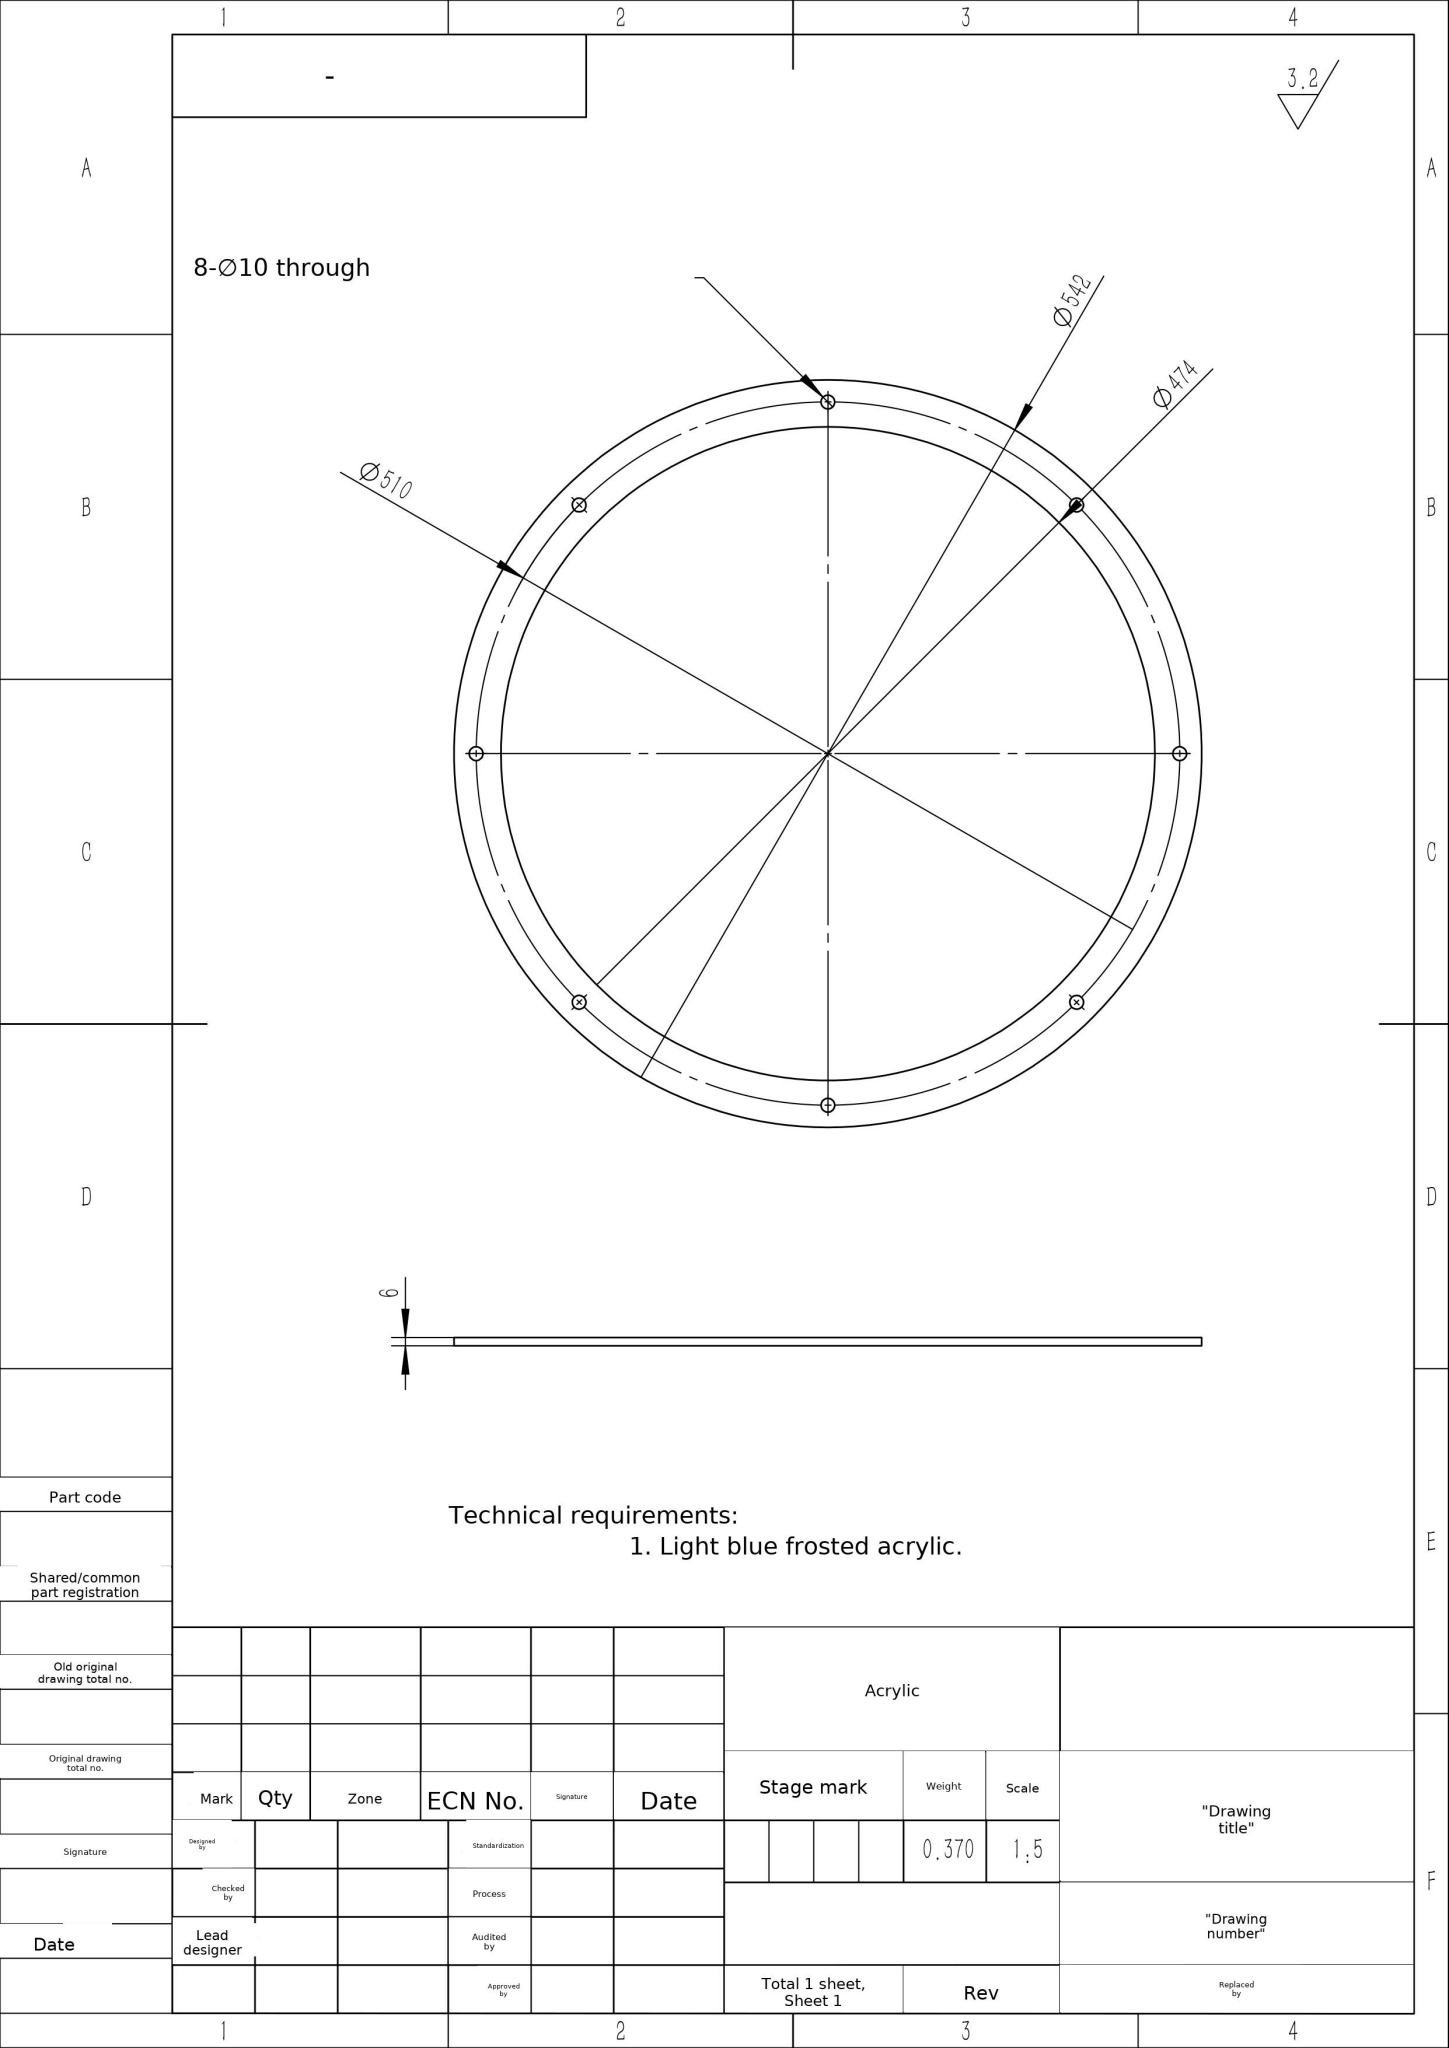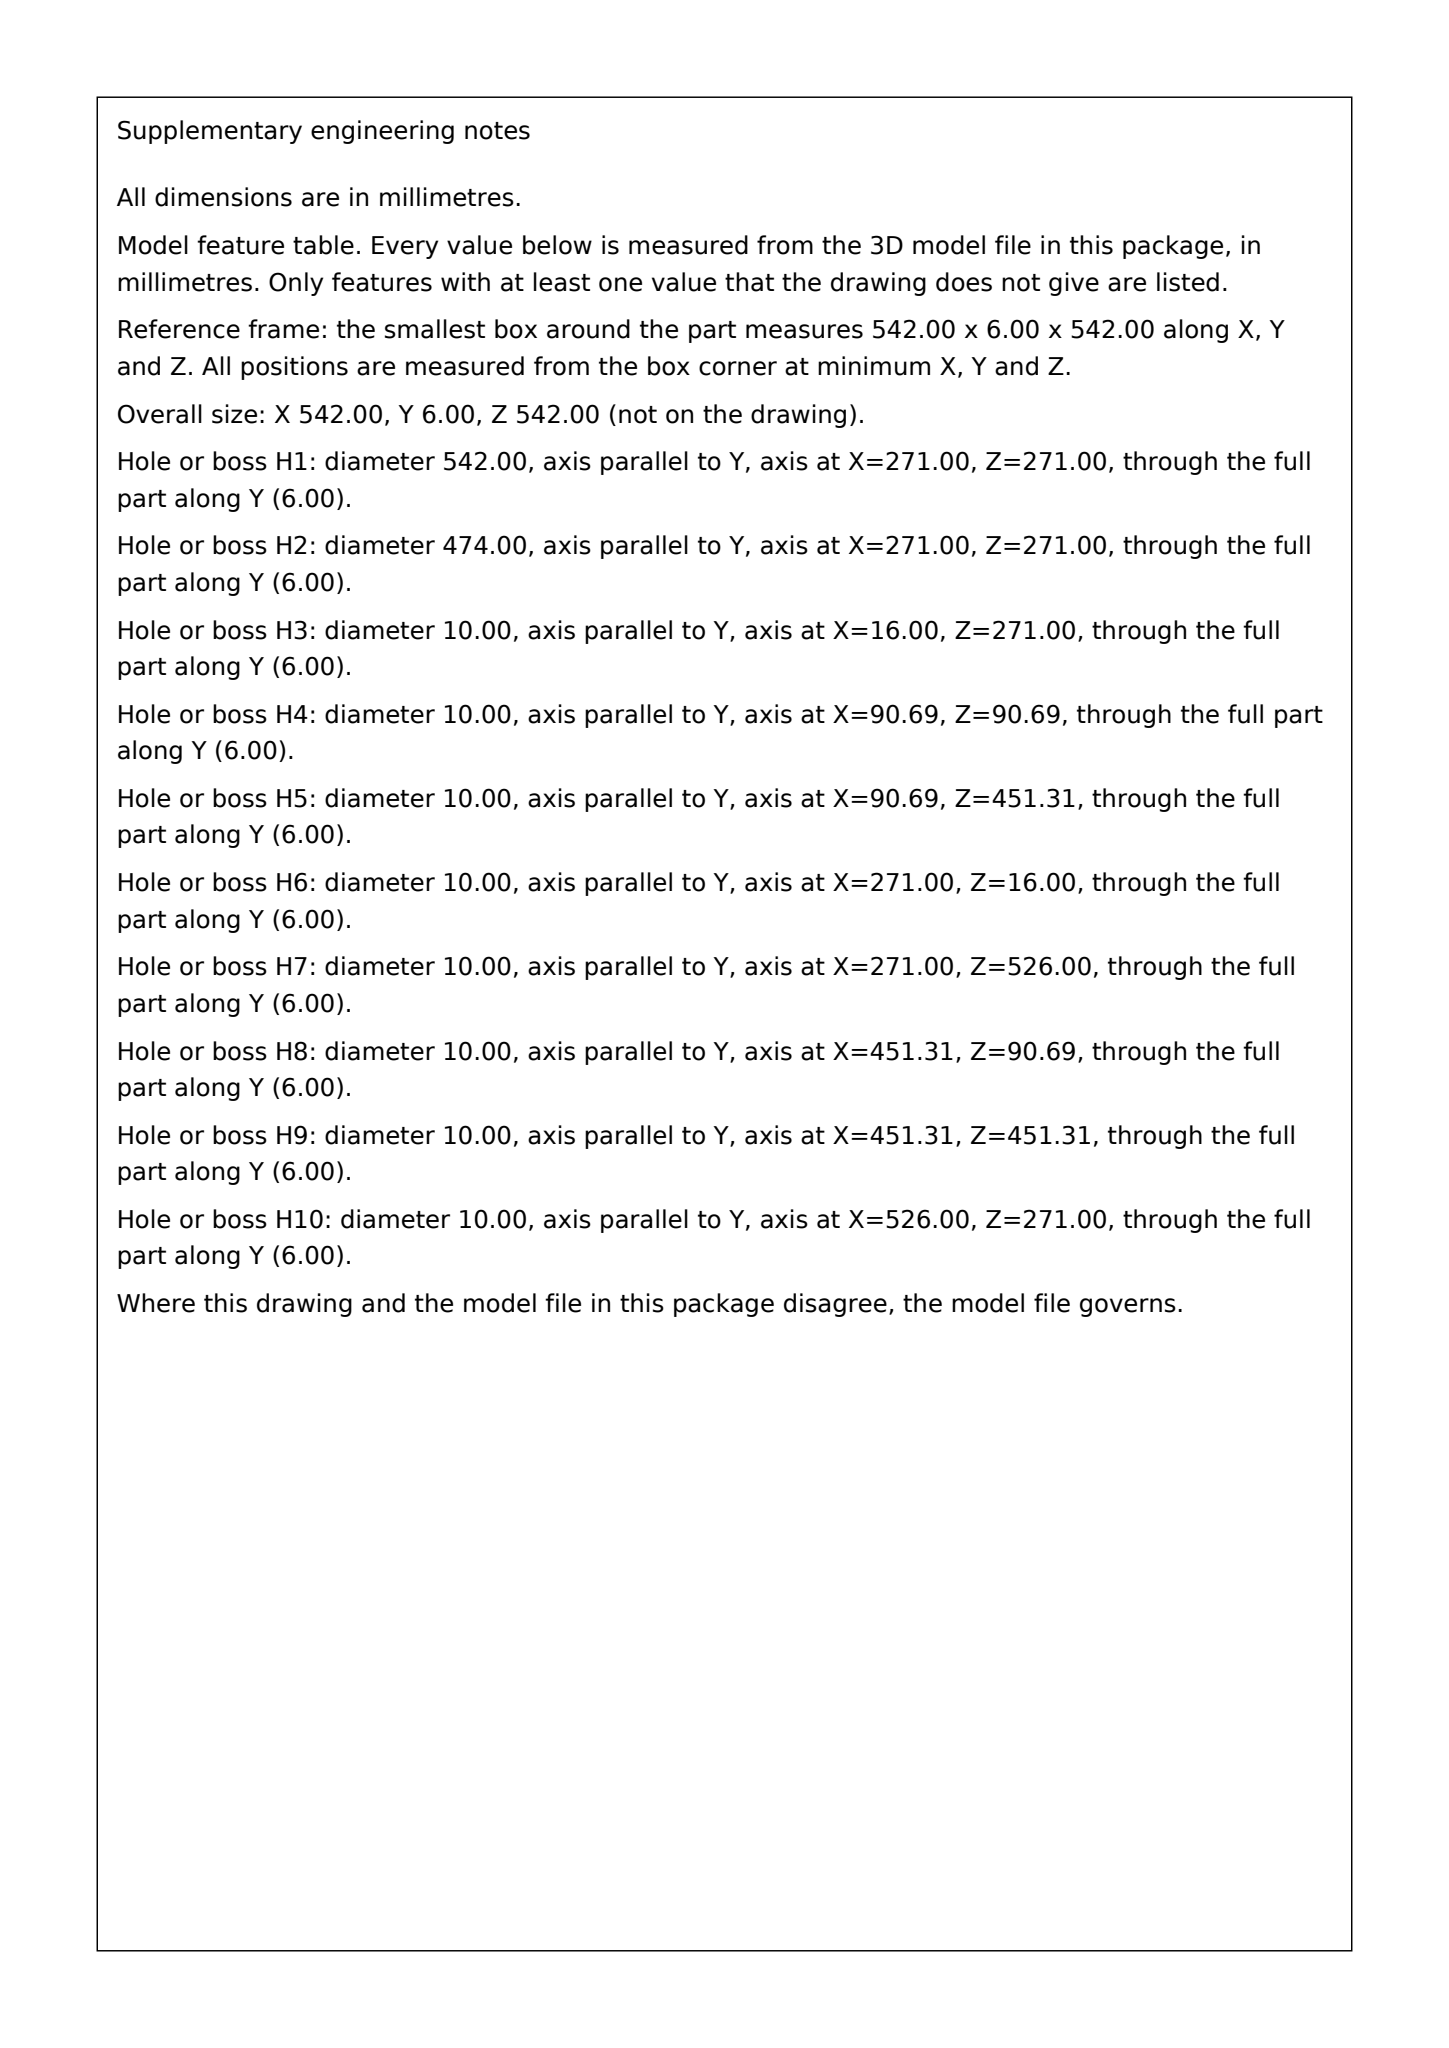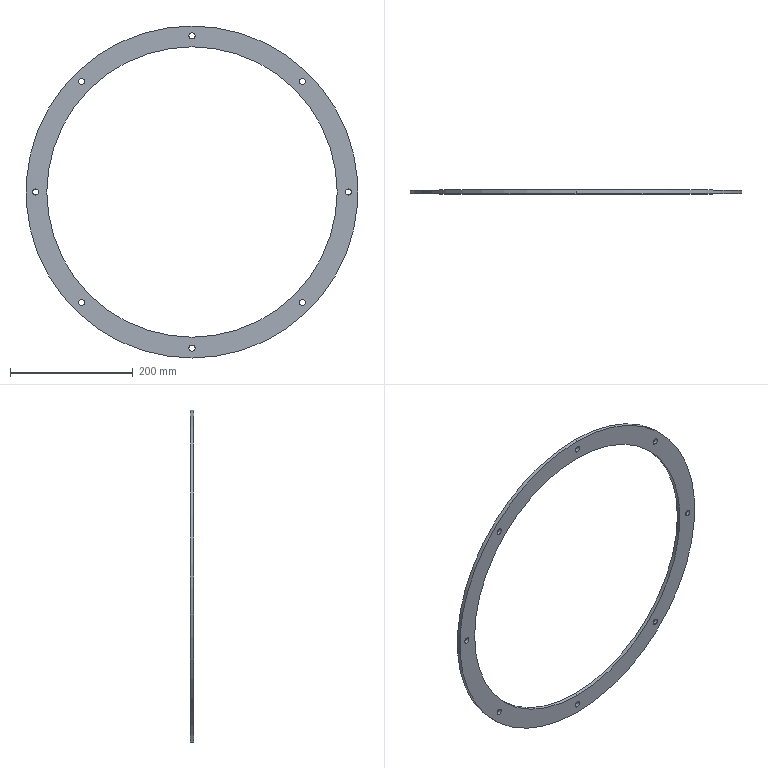Part | SolidWorks | mm | material Acrylic | 1 solid | 22 faces | box 542 x 6 x 542 mm | volume 321800 mm3 | cylinder 20 | plane 2 | commonest cylinder face diameters 10 x16 542 x2 474 x2
build123d program:
from build123d import *

# Parameters (mm, degrees)
SKETCH1_W          = 34
SKETCH1_H          = 3
SKETCH2_R          = 5
CUT_EXTRUDE1_DEPTH = 30
CIRPATTERN1_COUNT  = 8


with BuildPart() as part:
    # Sketch1 → Revolve1 (revolve)
    with BuildSketch(Plane.XY, mode=Mode.PRIVATE) as revolve1_sk:
        with Locations((254, 1.5)):
            Rectangle(SKETCH1_W, SKETCH1_H)
    revolve1 = revolve(revolve1_sk.sketch.rotate(Axis((0, 0, 0), (0, 1, 0)), 90), axis=Axis((0, 0, 0), (0, 1, 0)))


with BuildPart() as mirror1_1:
    # Mirror1: Revolve1 across Top Plane
    add(revolve1.mirror(Plane(origin=(0, 0, 0), x_dir=(1, 0, 0), z_dir=(0, 1, 0))))


with BuildPart() as part_1:
    add(part.part)

    # Mirror1 united with what the copies touc: union Mirror1_1
    add(mirror1_1.part)

    # Sketch2 → Cut-Extrude1 (cut)
    with BuildSketch(Plane(origin=(0, 3, 0), x_dir=(1, 0, 0), z_dir=(0, 1, 0))):
        with Locations(Location((255, 0, 0), (0, 0, 270))):
            Circle(SKETCH2_R)
    cut_extrude1 = extrude(amount=-CUT_EXTRUDE1_DEPTH, mode=Mode.SUBTRACT)

    # CirPattern1: Cut-Extrude1 ×8 about axis
    cirpattern1_axis = Axis((0, 0, 0), (0, 1, 0))
    for i in range(1, CIRPATTERN1_COUNT):
        add(cut_extrude1.rotate(cirpattern1_axis, i * 360 / CIRPATTERN1_COUNT), mode=Mode.SUBTRACT)


solid = part_1.part
STEP:
#1=CARTESIAN_POINT('',(-0.,-3.,250.));
#2=VERTEX_POINT('',#1);
#3=CARTESIAN_POINT('',(-0.,-3.,260.));
#4=VERTEX_POINT('',#3);
#5=CARTESIAN_POINT('',(-0.,-3.,255.));
#6=DIRECTION('',(0.,1.,0.));
#7=DIRECTION('',(0.,0.,1.));
#8=AXIS2_PLACEMENT_3D('',#5,#6,#7);
#9=CIRCLE('',#8,5.);
#10=EDGE_CURVE('',#2,#4,#9,.T.);
#11=ORIENTED_EDGE('',*,*,#10,.F.);
#12=CARTESIAN_POINT('',(-0.,3.,250.));
#13=VERTEX_POINT('',#12);
#14=CARTESIAN_POINT('',(-0.,-27.,250.));
#15=DIRECTION('',(0.,1.,0.));
#16=VECTOR('',#15,1000.);
#17=LINE('',#14,#16);
#18=EDGE_CURVE('',#2,#13,#17,.T.);
#19=ORIENTED_EDGE('',*,*,#18,.T.);
#20=CARTESIAN_POINT('',(-0.,3.,260.));
#21=VERTEX_POINT('',#20);
#22=CARTESIAN_POINT('',(-0.,3.,255.));
#23=DIRECTION('',(0.,1.,0.));
#24=DIRECTION('',(-1.,0.,0.));
#25=AXIS2_PLACEMENT_3D('',#22,#23,#24);
#26=CIRCLE('',#25,5.);
#27=EDGE_CURVE('',#13,#21,#26,.T.);
#28=ORIENTED_EDGE('',*,*,#27,.T.);
#29=CARTESIAN_POINT('',(-0.,-27.,260.));
#30=DIRECTION('',(0.,1.,0.));
#31=VECTOR('',#30,1000.);
#32=LINE('',#29,#31);
#33=EDGE_CURVE('',#4,#21,#32,.T.);
#34=ORIENTED_EDGE('',*,*,#33,.F.);
#35=EDGE_LOOP('',(#11,#19,#28,#34));
#36=FACE_OUTER_BOUND('',#35,.T.);
#37=CARTESIAN_POINT('',(-0.,-27.,255.));
#38=DIRECTION('',(0.,1.,0.));
#39=DIRECTION('',(0.,0.,1.));
#40=AXIS2_PLACEMENT_3D('',#37,#38,#39);
#41=CYLINDRICAL_SURFACE('',#40,5.);
#42=ADVANCED_FACE('',(#36),#41,.F.);
#43=CARTESIAN_POINT('',(-180.312,-3.,175.312));
#44=VERTEX_POINT('',#43);
#45=CARTESIAN_POINT('',(-180.312,-3.,185.312));
#46=VERTEX_POINT('',#45);
#47=CARTESIAN_POINT('',(-180.312,-3.,180.312));
#48=DIRECTION('',(0.,1.,0.));
#49=DIRECTION('',(0.,0.,1.));
#50=AXIS2_PLACEMENT_3D('',#47,#48,#49);
#51=CIRCLE('',#50,5.);
#52=EDGE_CURVE('',#44,#46,#51,.T.);
#53=ORIENTED_EDGE('',*,*,#52,.F.);
#54=CARTESIAN_POINT('',(-180.312,3.,175.312));
#55=VERTEX_POINT('',#54);
#56=CARTESIAN_POINT('',(-180.312,-27.,175.312));
#57=DIRECTION('',(0.,1.,0.));
#58=VECTOR('',#57,1000.);
#59=LINE('',#56,#58);
#60=EDGE_CURVE('',#44,#55,#59,.T.);
#61=ORIENTED_EDGE('',*,*,#60,.T.);
#62=CARTESIAN_POINT('',(-180.312,3.,185.312));
#63=VERTEX_POINT('',#62);
#64=CARTESIAN_POINT('',(-180.312,3.,180.312));
#65=DIRECTION('',(0.,1.,0.));
#66=DIRECTION('',(-0.7071,0.,-0.7071));
#67=AXIS2_PLACEMENT_3D('',#64,#65,#66);
#68=CIRCLE('',#67,5.);
#69=EDGE_CURVE('',#55,#63,#68,.T.);
#70=ORIENTED_EDGE('',*,*,#69,.T.);
#71=CARTESIAN_POINT('',(-180.312,-27.,185.312));
#72=DIRECTION('',(0.,1.,0.));
#73=VECTOR('',#72,1000.);
#74=LINE('',#71,#73);
#75=EDGE_CURVE('',#46,#63,#74,.T.);
#76=ORIENTED_EDGE('',*,*,#75,.F.);
#77=EDGE_LOOP('',(#53,#61,#70,#76));
#78=FACE_OUTER_BOUND('',#77,.T.);
#79=CARTESIAN_POINT('',(-180.312,-27.,180.312));
#80=DIRECTION('',(0.,1.,0.));
#81=DIRECTION('',(0.,0.,1.));
#82=AXIS2_PLACEMENT_3D('',#79,#80,#81);
#83=CYLINDRICAL_SURFACE('',#82,5.);
#84=ADVANCED_FACE('',(#78),#83,.F.);
#85=CARTESIAN_POINT('',(-255.,-3.,-5.));
#86=VERTEX_POINT('',#85);
#87=CARTESIAN_POINT('',(-255.,-3.,5.));
#88=VERTEX_POINT('',#87);
#89=CARTESIAN_POINT('',(-255.,-3.,0.));
#90=DIRECTION('',(0.,1.,0.));
#91=DIRECTION('',(0.,0.,1.));
#92=AXIS2_PLACEMENT_3D('',#89,#90,#91);
#93=CIRCLE('',#92,5.);
#94=EDGE_CURVE('',#86,#88,#93,.T.);
#95=ORIENTED_EDGE('',*,*,#94,.F.);
#96=CARTESIAN_POINT('',(-255.,3.,-5.));
#97=VERTEX_POINT('',#96);
#98=CARTESIAN_POINT('',(-255.,-27.,-5.));
#99=DIRECTION('',(0.,1.,0.));
#100=VECTOR('',#99,1000.);
#101=LINE('',#98,#100);
#102=EDGE_CURVE('',#86,#97,#101,.T.);
#103=ORIENTED_EDGE('',*,*,#102,.T.);
#104=CARTESIAN_POINT('',(-255.,3.,5.));
#105=VERTEX_POINT('',#104);
#106=CARTESIAN_POINT('',(-255.,3.,0.));
#107=DIRECTION('',(0.,1.,0.));
#108=DIRECTION('',(0.,0.,-1.));
#109=AXIS2_PLACEMENT_3D('',#106,#107,#108);
#110=CIRCLE('',#109,5.);
#111=EDGE_CURVE('',#97,#105,#110,.T.);
#112=ORIENTED_EDGE('',*,*,#111,.T.);
#113=CARTESIAN_POINT('',(-255.,-27.,5.));
#114=DIRECTION('',(0.,1.,0.));
#115=VECTOR('',#114,1000.);
#116=LINE('',#113,#115);
#117=EDGE_CURVE('',#88,#105,#116,.T.);
#118=ORIENTED_EDGE('',*,*,#117,.F.);
#119=EDGE_LOOP('',(#95,#103,#112,#118));
#120=FACE_OUTER_BOUND('',#119,.T.);
#121=CARTESIAN_POINT('',(-255.,-27.,0.));
#122=DIRECTION('',(0.,1.,0.));
#123=DIRECTION('',(0.,0.,1.));
#124=AXIS2_PLACEMENT_3D('',#121,#122,#123);
#125=CYLINDRICAL_SURFACE('',#124,5.);
#126=ADVANCED_FACE('',(#120),#125,.F.);
#127=CARTESIAN_POINT('',(-180.312,-3.,-185.312));
#128=VERTEX_POINT('',#127);
#129=CARTESIAN_POINT('',(-180.312,-3.,-175.312));
#130=VERTEX_POINT('',#129);
#131=CARTESIAN_POINT('',(-180.312,-3.,-180.312));
#132=DIRECTION('',(0.,1.,0.));
#133=DIRECTION('',(0.,0.,1.));
#134=AXIS2_PLACEMENT_3D('',#131,#132,#133);
#135=CIRCLE('',#134,5.);
#136=EDGE_CURVE('',#128,#130,#135,.T.);
#137=ORIENTED_EDGE('',*,*,#136,.F.);
#138=CARTESIAN_POINT('',(-180.312,3.,-185.312));
#139=VERTEX_POINT('',#138);
#140=CARTESIAN_POINT('',(-180.312,-27.,-185.312));
#141=DIRECTION('',(0.,1.,0.));
#142=VECTOR('',#141,1000.);
#143=LINE('',#140,#142);
#144=EDGE_CURVE('',#128,#139,#143,.T.);
#145=ORIENTED_EDGE('',*,*,#144,.T.);
#146=CARTESIAN_POINT('',(-180.312,3.,-175.312));
#147=VERTEX_POINT('',#146);
#148=CARTESIAN_POINT('',(-180.312,3.,-180.312));
#149=DIRECTION('',(0.,1.,0.));
#150=DIRECTION('',(0.7071,0.,-0.7071));
#151=AXIS2_PLACEMENT_3D('',#148,#149,#150);
#152=CIRCLE('',#151,5.);
#153=EDGE_CURVE('',#139,#147,#152,.T.);
#154=ORIENTED_EDGE('',*,*,#153,.T.);
#155=CARTESIAN_POINT('',(-180.312,-27.,-175.312));
#156=DIRECTION('',(0.,1.,0.));
#157=VECTOR('',#156,1000.);
#158=LINE('',#155,#157);
#159=EDGE_CURVE('',#130,#147,#158,.T.);
#160=ORIENTED_EDGE('',*,*,#159,.F.);
#161=EDGE_LOOP('',(#137,#145,#154,#160));
#162=FACE_OUTER_BOUND('',#161,.T.);
#163=CARTESIAN_POINT('',(-180.312,-27.,-180.312));
#164=DIRECTION('',(0.,1.,0.));
#165=DIRECTION('',(0.,0.,1.));
#166=AXIS2_PLACEMENT_3D('',#163,#164,#165);
#167=CYLINDRICAL_SURFACE('',#166,5.);
#168=ADVANCED_FACE('',(#162),#167,.F.);
#169=CARTESIAN_POINT('',(0.,-3.,-260.));
#170=VERTEX_POINT('',#169);
#171=CARTESIAN_POINT('',(0.,-3.,-250.));
#172=VERTEX_POINT('',#171);
#173=CARTESIAN_POINT('',(0.,-3.,-255.));
#174=DIRECTION('',(0.,1.,0.));
#175=DIRECTION('',(0.,0.,1.));
#176=AXIS2_PLACEMENT_3D('',#173,#174,#175);
#177=CIRCLE('',#176,5.);
#178=EDGE_CURVE('',#170,#172,#177,.T.);
#179=ORIENTED_EDGE('',*,*,#178,.F.);
#180=CARTESIAN_POINT('',(0.,3.,-260.));
#181=VERTEX_POINT('',#180);
#182=CARTESIAN_POINT('',(0.,-27.,-260.));
#183=DIRECTION('',(0.,1.,0.));
#184=VECTOR('',#183,1000.);
#185=LINE('',#182,#184);
#186=EDGE_CURVE('',#170,#181,#185,.T.);
#187=ORIENTED_EDGE('',*,*,#186,.T.);
#188=CARTESIAN_POINT('',(0.,3.,-250.));
#189=VERTEX_POINT('',#188);
#190=CARTESIAN_POINT('',(0.,3.,-255.));
#191=DIRECTION('',(0.,1.,0.));
#192=DIRECTION('',(1.,0.,0.));
#193=AXIS2_PLACEMENT_3D('',#190,#191,#192);
#194=CIRCLE('',#193,5.);
#195=EDGE_CURVE('',#181,#189,#194,.T.);
#196=ORIENTED_EDGE('',*,*,#195,.T.);
#197=CARTESIAN_POINT('',(0.,-27.,-250.));
#198=DIRECTION('',(0.,1.,0.));
#199=VECTOR('',#198,1000.);
#200=LINE('',#197,#199);
#201=EDGE_CURVE('',#172,#189,#200,.T.);
#202=ORIENTED_EDGE('',*,*,#201,.F.);
#203=EDGE_LOOP('',(#179,#187,#196,#202));
#204=FACE_OUTER_BOUND('',#203,.T.);
#205=CARTESIAN_POINT('',(0.,-27.,-255.));
#206=DIRECTION('',(0.,1.,0.));
#207=DIRECTION('',(0.,0.,1.));
#208=AXIS2_PLACEMENT_3D('',#205,#206,#207);
#209=CYLINDRICAL_SURFACE('',#208,5.);
#210=ADVANCED_FACE('',(#204),#209,.F.);
#211=CARTESIAN_POINT('',(180.312,-3.,-185.312));
#212=VERTEX_POINT('',#211);
#213=CARTESIAN_POINT('',(180.312,-3.,-175.312));
#214=VERTEX_POINT('',#213);
#215=CARTESIAN_POINT('',(180.312,-3.,-180.312));
#216=DIRECTION('',(0.,1.,0.));
#217=DIRECTION('',(0.,0.,1.));
#218=AXIS2_PLACEMENT_3D('',#215,#216,#217);
#219=CIRCLE('',#218,5.);
#220=EDGE_CURVE('',#212,#214,#219,.T.);
#221=ORIENTED_EDGE('',*,*,#220,.F.);
#222=CARTESIAN_POINT('',(180.312,3.,-185.312));
#223=VERTEX_POINT('',#222);
#224=CARTESIAN_POINT('',(180.312,-27.,-185.312));
#225=DIRECTION('',(0.,1.,0.));
#226=VECTOR('',#225,1000.);
#227=LINE('',#224,#226);
#228=EDGE_CURVE('',#212,#223,#227,.T.);
#229=ORIENTED_EDGE('',*,*,#228,.T.);
#230=CARTESIAN_POINT('',(180.312,3.,-175.312));
#231=VERTEX_POINT('',#230);
#232=CARTESIAN_POINT('',(180.312,3.,-180.312));
#233=DIRECTION('',(0.,1.,0.));
#234=DIRECTION('',(0.7071,0.,0.7071));
#235=AXIS2_PLACEMENT_3D('',#232,#233,#234);
#236=CIRCLE('',#235,5.);
#237=EDGE_CURVE('',#223,#231,#236,.T.);
#238=ORIENTED_EDGE('',*,*,#237,.T.);
#239=CARTESIAN_POINT('',(180.312,-27.,-175.312));
#240=DIRECTION('',(0.,1.,0.));
#241=VECTOR('',#240,1000.);
#242=LINE('',#239,#241);
#243=EDGE_CURVE('',#214,#231,#242,.T.);
#244=ORIENTED_EDGE('',*,*,#243,.F.);
#245=EDGE_LOOP('',(#221,#229,#238,#244));
#246=FACE_OUTER_BOUND('',#245,.T.);
#247=CARTESIAN_POINT('',(180.312,-27.,-180.312));
#248=DIRECTION('',(0.,1.,0.));
#249=DIRECTION('',(0.,0.,1.));
#250=AXIS2_PLACEMENT_3D('',#247,#248,#249);
#251=CYLINDRICAL_SURFACE('',#250,5.);
#252=ADVANCED_FACE('',(#246),#251,.F.);
#253=CARTESIAN_POINT('',(180.312,-3.,175.312));
#254=VERTEX_POINT('',#253);
#255=CARTESIAN_POINT('',(180.312,-3.,185.312));
#256=VERTEX_POINT('',#255);
#257=CARTESIAN_POINT('',(180.312,-3.,180.312));
#258=DIRECTION('',(0.,1.,0.));
#259=DIRECTION('',(0.,0.,1.));
#260=AXIS2_PLACEMENT_3D('',#257,#258,#259);
#261=CIRCLE('',#260,5.);
#262=EDGE_CURVE('',#254,#256,#261,.T.);
#263=ORIENTED_EDGE('',*,*,#262,.F.);
#264=CARTESIAN_POINT('',(180.312,3.,175.312));
#265=VERTEX_POINT('',#264);
#266=CARTESIAN_POINT('',(180.312,-27.,175.312));
#267=DIRECTION('',(0.,1.,0.));
#268=VECTOR('',#267,1000.);
#269=LINE('',#266,#268);
#270=EDGE_CURVE('',#254,#265,#269,.T.);
#271=ORIENTED_EDGE('',*,*,#270,.T.);
#272=CARTESIAN_POINT('',(180.312,3.,185.312));
#273=VERTEX_POINT('',#272);
#274=CARTESIAN_POINT('',(180.312,3.,180.312));
#275=DIRECTION('',(0.,1.,0.));
#276=DIRECTION('',(-0.7071,0.,0.7071));
#277=AXIS2_PLACEMENT_3D('',#274,#275,#276);
#278=CIRCLE('',#277,5.);
#279=EDGE_CURVE('',#265,#273,#278,.T.);
#280=ORIENTED_EDGE('',*,*,#279,.T.);
#281=CARTESIAN_POINT('',(180.312,-27.,185.312));
#282=DIRECTION('',(0.,1.,0.));
#283=VECTOR('',#282,1000.);
#284=LINE('',#281,#283);
#285=EDGE_CURVE('',#256,#273,#284,.T.);
#286=ORIENTED_EDGE('',*,*,#285,.F.);
#287=EDGE_LOOP('',(#263,#271,#280,#286));
#288=FACE_OUTER_BOUND('',#287,.T.);
#289=CARTESIAN_POINT('',(180.312,-27.,180.312));
#290=DIRECTION('',(0.,1.,0.));
#291=DIRECTION('',(0.,0.,1.));
#292=AXIS2_PLACEMENT_3D('',#289,#290,#291);
#293=CYLINDRICAL_SURFACE('',#292,5.);
#294=ADVANCED_FACE('',(#288),#293,.F.);
#295=CARTESIAN_POINT('',(255.,-3.,-5.));
#296=VERTEX_POINT('',#295);
#297=CARTESIAN_POINT('',(255.,-3.,5.));
#298=VERTEX_POINT('',#297);
#299=CARTESIAN_POINT('',(255.,-3.,0.));
#300=DIRECTION('',(0.,1.,0.));
#301=DIRECTION('',(0.,0.,1.));
#302=AXIS2_PLACEMENT_3D('',#299,#300,#301);
#303=CIRCLE('',#302,5.);
#304=EDGE_CURVE('',#296,#298,#303,.T.);
#305=ORIENTED_EDGE('',*,*,#304,.F.);
#306=CARTESIAN_POINT('',(255.,3.,-5.));
#307=VERTEX_POINT('',#306);
#308=CARTESIAN_POINT('',(255.,-27.,-5.));
#309=DIRECTION('',(0.,1.,0.));
#310=VECTOR('',#309,1000.);
#311=LINE('',#308,#310);
#312=EDGE_CURVE('',#296,#307,#311,.T.);
#313=ORIENTED_EDGE('',*,*,#312,.T.);
#314=CARTESIAN_POINT('',(255.,3.,5.));
#315=VERTEX_POINT('',#314);
#316=CARTESIAN_POINT('',(255.,3.,0.));
#317=DIRECTION('',(0.,1.,0.));
#318=DIRECTION('',(0.,0.,1.));
#319=AXIS2_PLACEMENT_3D('',#316,#317,#318);
#320=CIRCLE('',#319,5.);
#321=EDGE_CURVE('',#307,#315,#320,.T.);
#322=ORIENTED_EDGE('',*,*,#321,.T.);
#323=CARTESIAN_POINT('',(255.,-27.,5.));
#324=DIRECTION('',(0.,1.,0.));
#325=VECTOR('',#324,1000.);
#326=LINE('',#323,#325);
#327=EDGE_CURVE('',#298,#315,#326,.T.);
#328=ORIENTED_EDGE('',*,*,#327,.F.);
#329=EDGE_LOOP('',(#305,#313,#322,#328));
#330=FACE_OUTER_BOUND('',#329,.T.);
#331=CARTESIAN_POINT('',(255.,-27.,0.));
#332=DIRECTION('',(0.,1.,0.));
#333=DIRECTION('',(0.,0.,1.));
#334=AXIS2_PLACEMENT_3D('',#331,#332,#333);
#335=CYLINDRICAL_SURFACE('',#334,5.);
#336=ADVANCED_FACE('',(#330),#335,.F.);
#337=CARTESIAN_POINT('',(0.,3.,-271.));
#338=VERTEX_POINT('',#337);
#339=CARTESIAN_POINT('',(0.,3.,271.));
#340=VERTEX_POINT('',#339);
#341=CARTESIAN_POINT('',(0.,3.,0.));
#342=DIRECTION('',(0.,-1.,0.));
#343=DIRECTION('',(0.,0.,-1.));
#344=AXIS2_PLACEMENT_3D('',#341,#342,#343);
#345=CIRCLE('',#344,271.);
#346=EDGE_CURVE('',#338,#340,#345,.T.);
#347=ORIENTED_EDGE('',*,*,#346,.T.);
#348=CARTESIAN_POINT('',(0.,-3.,271.));
#349=VERTEX_POINT('',#348);
#350=CARTESIAN_POINT('',(0.,0.,271.));
#351=DIRECTION('',(0.,-1.,0.));
#352=VECTOR('',#351,1000.);
#353=LINE('',#350,#352);
#354=EDGE_CURVE('',#340,#349,#353,.T.);
#355=ORIENTED_EDGE('',*,*,#354,.T.);
#356=CARTESIAN_POINT('',(0.,-3.,-271.));
#357=VERTEX_POINT('',#356);
#358=CARTESIAN_POINT('',(0.,-3.,0.));
#359=DIRECTION('',(0.,-1.,0.));
#360=DIRECTION('',(0.,0.,-1.));
#361=AXIS2_PLACEMENT_3D('',#358,#359,#360);
#362=CIRCLE('',#361,271.);
#363=EDGE_CURVE('',#357,#349,#362,.T.);
#364=ORIENTED_EDGE('',*,*,#363,.F.);
#365=CARTESIAN_POINT('',(0.,0.,-271.));
#366=DIRECTION('',(0.,-1.,0.));
#367=VECTOR('',#366,1000.);
#368=LINE('',#365,#367);
#369=EDGE_CURVE('',#338,#357,#368,.T.);
#370=ORIENTED_EDGE('',*,*,#369,.F.);
#371=EDGE_LOOP('',(#347,#355,#364,#370));
#372=FACE_OUTER_BOUND('',#371,.T.);
#373=CARTESIAN_POINT('',(0.,0.,0.));
#374=DIRECTION('',(0.,-1.,0.));
#375=DIRECTION('',(0.,0.,-1.));
#376=AXIS2_PLACEMENT_3D('',#373,#374,#375);
#377=CYLINDRICAL_SURFACE('',#376,271.);
#378=ADVANCED_FACE('',(#372),#377,.T.);
#379=CARTESIAN_POINT('',(0.,3.,237.));
#380=VERTEX_POINT('',#379);
#381=CARTESIAN_POINT('',(0.,3.,-237.));
#382=VERTEX_POINT('',#381);
#383=CARTESIAN_POINT('',(0.,3.,0.));
#384=DIRECTION('',(0.,-1.,0.));
#385=DIRECTION('',(0.,0.,-1.));
#386=AXIS2_PLACEMENT_3D('',#383,#384,#385);
#387=CIRCLE('',#386,237.);
#388=EDGE_CURVE('',#380,#382,#387,.T.);
#389=ORIENTED_EDGE('',*,*,#388,.F.);
#390=CARTESIAN_POINT('',(0.,-3.,237.));
#391=VERTEX_POINT('',#390);
#392=CARTESIAN_POINT('',(0.,0.,237.));
#393=DIRECTION('',(0.,-1.,0.));
#394=VECTOR('',#393,1000.);
#395=LINE('',#392,#394);
#396=EDGE_CURVE('',#380,#391,#395,.T.);
#397=ORIENTED_EDGE('',*,*,#396,.T.);
#398=CARTESIAN_POINT('',(0.,-3.,-237.));
#399=VERTEX_POINT('',#398);
#400=CARTESIAN_POINT('',(0.,-3.,0.));
#401=DIRECTION('',(0.,-1.,0.));
#402=DIRECTION('',(0.,0.,-1.));
#403=AXIS2_PLACEMENT_3D('',#400,#401,#402);
#404=CIRCLE('',#403,237.);
#405=EDGE_CURVE('',#391,#399,#404,.T.);
#406=ORIENTED_EDGE('',*,*,#405,.T.);
#407=CARTESIAN_POINT('',(0.,0.,-237.));
#408=DIRECTION('',(0.,-1.,0.));
#409=VECTOR('',#408,1000.);
#410=LINE('',#407,#409);
#411=EDGE_CURVE('',#382,#399,#410,.T.);
#412=ORIENTED_EDGE('',*,*,#411,.F.);
#413=EDGE_LOOP('',(#389,#397,#406,#412));
#414=FACE_OUTER_BOUND('',#413,.T.);
#415=CARTESIAN_POINT('',(0.,0.,0.));
#416=DIRECTION('',(0.,-1.,0.));
#417=DIRECTION('',(0.,0.,-1.));
#418=AXIS2_PLACEMENT_3D('',#415,#416,#417);
#419=CYLINDRICAL_SURFACE('',#418,237.);
#420=ADVANCED_FACE('',(#414),#419,.F.);
#421=CARTESIAN_POINT('',(-0.,3.,255.));
#422=DIRECTION('',(0.,1.,0.));
#423=DIRECTION('',(-1.,0.,0.));
#424=AXIS2_PLACEMENT_3D('',#421,#422,#423);
#425=CIRCLE('',#424,5.);
#426=EDGE_CURVE('',#21,#13,#425,.T.);
#427=ORIENTED_EDGE('',*,*,#426,.F.);
#428=ORIENTED_EDGE('',*,*,#27,.F.);
#429=EDGE_LOOP('',(#427,#428));
#430=FACE_BOUND('',#429,.T.);
#431=CARTESIAN_POINT('',(-180.312,3.,180.312));
#432=DIRECTION('',(0.,1.,0.));
#433=DIRECTION('',(-0.7071,0.,-0.7071));
#434=AXIS2_PLACEMENT_3D('',#431,#432,#433);
#435=CIRCLE('',#434,5.);
#436=EDGE_CURVE('',#63,#55,#435,.T.);
#437=ORIENTED_EDGE('',*,*,#436,.F.);
#438=ORIENTED_EDGE('',*,*,#69,.F.);
#439=EDGE_LOOP('',(#437,#438));
#440=FACE_BOUND('',#439,.T.);
#441=CARTESIAN_POINT('',(-255.,3.,0.));
#442=DIRECTION('',(0.,1.,0.));
#443=DIRECTION('',(0.,0.,-1.));
#444=AXIS2_PLACEMENT_3D('',#441,#442,#443);
#445=CIRCLE('',#444,5.);
#446=EDGE_CURVE('',#105,#97,#445,.T.);
#447=ORIENTED_EDGE('',*,*,#446,.F.);
#448=ORIENTED_EDGE('',*,*,#111,.F.);
#449=EDGE_LOOP('',(#447,#448));
#450=FACE_BOUND('',#449,.T.);
#451=CARTESIAN_POINT('',(-180.312,3.,-180.312));
#452=DIRECTION('',(0.,1.,0.));
#453=DIRECTION('',(0.7071,0.,-0.7071));
#454=AXIS2_PLACEMENT_3D('',#451,#452,#453);
#455=CIRCLE('',#454,5.);
#456=EDGE_CURVE('',#147,#139,#455,.T.);
#457=ORIENTED_EDGE('',*,*,#456,.F.);
#458=ORIENTED_EDGE('',*,*,#153,.F.);
#459=EDGE_LOOP('',(#457,#458));
#460=FACE_BOUND('',#459,.T.);
#461=CARTESIAN_POINT('',(0.,3.,-255.));
#462=DIRECTION('',(0.,1.,0.));
#463=DIRECTION('',(1.,0.,0.));
#464=AXIS2_PLACEMENT_3D('',#461,#462,#463);
#465=CIRCLE('',#464,5.);
#466=EDGE_CURVE('',#189,#181,#465,.T.);
#467=ORIENTED_EDGE('',*,*,#466,.F.);
#468=ORIENTED_EDGE('',*,*,#195,.F.);
#469=EDGE_LOOP('',(#467,#468));
#470=FACE_BOUND('',#469,.T.);
#471=CARTESIAN_POINT('',(180.312,3.,-180.312));
#472=DIRECTION('',(0.,1.,0.));
#473=DIRECTION('',(0.7071,0.,0.7071));
#474=AXIS2_PLACEMENT_3D('',#471,#472,#473);
#475=CIRCLE('',#474,5.);
#476=EDGE_CURVE('',#231,#223,#475,.T.);
#477=ORIENTED_EDGE('',*,*,#476,.F.);
#478=ORIENTED_EDGE('',*,*,#237,.F.);
#479=EDGE_LOOP('',(#477,#478));
#480=FACE_BOUND('',#479,.T.);
#481=CARTESIAN_POINT('',(180.312,3.,180.312));
#482=DIRECTION('',(0.,1.,0.));
#483=DIRECTION('',(-0.7071,0.,0.7071));
#484=AXIS2_PLACEMENT_3D('',#481,#482,#483);
#485=CIRCLE('',#484,5.);
#486=EDGE_CURVE('',#273,#265,#485,.T.);
#487=ORIENTED_EDGE('',*,*,#486,.F.);
#488=ORIENTED_EDGE('',*,*,#279,.F.);
#489=EDGE_LOOP('',(#487,#488));
#490=FACE_BOUND('',#489,.T.);
#491=CARTESIAN_POINT('',(255.,3.,0.));
#492=DIRECTION('',(0.,1.,0.));
#493=DIRECTION('',(0.,0.,1.));
#494=AXIS2_PLACEMENT_3D('',#491,#492,#493);
#495=CIRCLE('',#494,5.);
#496=EDGE_CURVE('',#315,#307,#495,.T.);
#497=ORIENTED_EDGE('',*,*,#496,.F.);
#498=ORIENTED_EDGE('',*,*,#321,.F.);
#499=EDGE_LOOP('',(#497,#498));
#500=FACE_BOUND('',#499,.T.);
#501=ORIENTED_EDGE('',*,*,#346,.F.);
#502=CARTESIAN_POINT('',(0.,3.,0.));
#503=DIRECTION('',(0.,-1.,0.));
#504=DIRECTION('',(0.,0.,-1.));
#505=AXIS2_PLACEMENT_3D('',#502,#503,#504);
#506=CIRCLE('',#505,271.);
#507=EDGE_CURVE('',#340,#338,#506,.T.);
#508=ORIENTED_EDGE('',*,*,#507,.F.);
#509=EDGE_LOOP('',(#501,#508));
#510=FACE_OUTER_BOUND('',#509,.T.);
#511=CARTESIAN_POINT('',(0.,3.,0.));
#512=DIRECTION('',(0.,-1.,0.));
#513=DIRECTION('',(0.,0.,-1.));
#514=AXIS2_PLACEMENT_3D('',#511,#512,#513);
#515=CIRCLE('',#514,237.);
#516=EDGE_CURVE('',#382,#380,#515,.T.);
#517=ORIENTED_EDGE('',*,*,#516,.T.);
#518=ORIENTED_EDGE('',*,*,#388,.T.);
#519=EDGE_LOOP('',(#517,#518));
#520=FACE_BOUND('',#519,.T.);
#521=CARTESIAN_POINT('',(0.,3.,0.));
#522=DIRECTION('',(0.,-1.,0.));
#523=DIRECTION('',(0.,0.,-1.));
#524=AXIS2_PLACEMENT_3D('',#521,#522,#523);
#525=PLANE('',#524);
#526=ADVANCED_FACE('',(#430,#440,#450,#460,#470,#480,#490,#500,#510,#520),#525,.F.);
#527=ORIENTED_EDGE('',*,*,#396,.F.);
#528=ORIENTED_EDGE('',*,*,#516,.F.);
#529=ORIENTED_EDGE('',*,*,#411,.T.);
#530=CARTESIAN_POINT('',(0.,-3.,0.));
#531=DIRECTION('',(0.,-1.,0.));
#532=DIRECTION('',(0.,0.,-1.));
#533=AXIS2_PLACEMENT_3D('',#530,#531,#532);
#534=CIRCLE('',#533,237.);
#535=EDGE_CURVE('',#399,#391,#534,.T.);
#536=ORIENTED_EDGE('',*,*,#535,.T.);
#537=EDGE_LOOP('',(#527,#528,#529,#536));
#538=FACE_OUTER_BOUND('',#537,.T.);
#539=CARTESIAN_POINT('',(0.,0.,0.));
#540=DIRECTION('',(0.,-1.,0.));
#541=DIRECTION('',(0.,0.,-1.));
#542=AXIS2_PLACEMENT_3D('',#539,#540,#541);
#543=CYLINDRICAL_SURFACE('',#542,237.);
#544=ADVANCED_FACE('',(#538),#543,.F.);
#545=ORIENTED_EDGE('',*,*,#354,.F.);
#546=ORIENTED_EDGE('',*,*,#507,.T.);
#547=ORIENTED_EDGE('',*,*,#369,.T.);
#548=CARTESIAN_POINT('',(0.,-3.,0.));
#549=DIRECTION('',(0.,-1.,0.));
#550=DIRECTION('',(0.,0.,-1.));
#551=AXIS2_PLACEMENT_3D('',#548,#549,#550);
#552=CIRCLE('',#551,271.);
#553=EDGE_CURVE('',#349,#357,#552,.T.);
#554=ORIENTED_EDGE('',*,*,#553,.F.);
#555=EDGE_LOOP('',(#545,#546,#547,#554));
#556=FACE_OUTER_BOUND('',#555,.T.);
#557=CARTESIAN_POINT('',(0.,0.,0.));
#558=DIRECTION('',(0.,-1.,0.));
#559=DIRECTION('',(0.,0.,-1.));
#560=AXIS2_PLACEMENT_3D('',#557,#558,#559);
#561=CYLINDRICAL_SURFACE('',#560,271.);
#562=ADVANCED_FACE('',(#556),#561,.T.);
#563=CARTESIAN_POINT('',(-0.,-3.,255.));
#564=DIRECTION('',(0.,1.,0.));
#565=DIRECTION('',(0.,0.,1.));
#566=AXIS2_PLACEMENT_3D('',#563,#564,#565);
#567=CIRCLE('',#566,5.);
#568=EDGE_CURVE('',#4,#2,#567,.T.);
#569=ORIENTED_EDGE('',*,*,#568,.T.);
#570=ORIENTED_EDGE('',*,*,#10,.T.);
#571=EDGE_LOOP('',(#569,#570));
#572=FACE_BOUND('',#571,.T.);
#573=CARTESIAN_POINT('',(-180.312,-3.,180.312));
#574=DIRECTION('',(0.,1.,0.));
#575=DIRECTION('',(0.,0.,1.));
#576=AXIS2_PLACEMENT_3D('',#573,#574,#575);
#577=CIRCLE('',#576,5.);
#578=EDGE_CURVE('',#46,#44,#577,.T.);
#579=ORIENTED_EDGE('',*,*,#578,.T.);
#580=ORIENTED_EDGE('',*,*,#52,.T.);
#581=EDGE_LOOP('',(#579,#580));
#582=FACE_BOUND('',#581,.T.);
#583=CARTESIAN_POINT('',(-255.,-3.,0.));
#584=DIRECTION('',(0.,1.,0.));
#585=DIRECTION('',(0.,0.,1.));
#586=AXIS2_PLACEMENT_3D('',#583,#584,#585);
#587=CIRCLE('',#586,5.);
#588=EDGE_CURVE('',#88,#86,#587,.T.);
#589=ORIENTED_EDGE('',*,*,#588,.T.);
#590=ORIENTED_EDGE('',*,*,#94,.T.);
#591=EDGE_LOOP('',(#589,#590));
#592=FACE_BOUND('',#591,.T.);
#593=CARTESIAN_POINT('',(-180.312,-3.,-180.312));
#594=DIRECTION('',(0.,1.,0.));
#595=DIRECTION('',(0.,0.,1.));
#596=AXIS2_PLACEMENT_3D('',#593,#594,#595);
#597=CIRCLE('',#596,5.);
#598=EDGE_CURVE('',#130,#128,#597,.T.);
#599=ORIENTED_EDGE('',*,*,#598,.T.);
#600=ORIENTED_EDGE('',*,*,#136,.T.);
#601=EDGE_LOOP('',(#599,#600));
#602=FACE_BOUND('',#601,.T.);
#603=CARTESIAN_POINT('',(0.,-3.,-255.));
#604=DIRECTION('',(0.,1.,0.));
#605=DIRECTION('',(0.,0.,1.));
#606=AXIS2_PLACEMENT_3D('',#603,#604,#605);
#607=CIRCLE('',#606,5.);
#608=EDGE_CURVE('',#172,#170,#607,.T.);
#609=ORIENTED_EDGE('',*,*,#608,.T.);
#610=ORIENTED_EDGE('',*,*,#178,.T.);
#611=EDGE_LOOP('',(#609,#610));
#612=FACE_BOUND('',#611,.T.);
#613=CARTESIAN_POINT('',(180.312,-3.,-180.312));
#614=DIRECTION('',(0.,1.,0.));
#615=DIRECTION('',(0.,0.,1.));
#616=AXIS2_PLACEMENT_3D('',#613,#614,#615);
#617=CIRCLE('',#616,5.);
#618=EDGE_CURVE('',#214,#212,#617,.T.);
#619=ORIENTED_EDGE('',*,*,#618,.T.);
#620=ORIENTED_EDGE('',*,*,#220,.T.);
#621=EDGE_LOOP('',(#619,#620));
#622=FACE_BOUND('',#621,.T.);
#623=CARTESIAN_POINT('',(180.312,-3.,180.312));
#624=DIRECTION('',(0.,1.,0.));
#625=DIRECTION('',(0.,0.,1.));
#626=AXIS2_PLACEMENT_3D('',#623,#624,#625);
#627=CIRCLE('',#626,5.);
#628=EDGE_CURVE('',#256,#254,#627,.T.);
#629=ORIENTED_EDGE('',*,*,#628,.T.);
#630=ORIENTED_EDGE('',*,*,#262,.T.);
#631=EDGE_LOOP('',(#629,#630));
#632=FACE_BOUND('',#631,.T.);
#633=CARTESIAN_POINT('',(255.,-3.,0.));
#634=DIRECTION('',(0.,1.,0.));
#635=DIRECTION('',(0.,0.,1.));
#636=AXIS2_PLACEMENT_3D('',#633,#634,#635);
#637=CIRCLE('',#636,5.);
#638=EDGE_CURVE('',#298,#296,#637,.T.);
#639=ORIENTED_EDGE('',*,*,#638,.T.);
#640=ORIENTED_EDGE('',*,*,#304,.T.);
#641=EDGE_LOOP('',(#639,#640));
#642=FACE_BOUND('',#641,.T.);
#643=ORIENTED_EDGE('',*,*,#363,.T.);
#644=ORIENTED_EDGE('',*,*,#553,.T.);
#645=EDGE_LOOP('',(#643,#644));
#646=FACE_OUTER_BOUND('',#645,.T.);
#647=ORIENTED_EDGE('',*,*,#535,.F.);
#648=ORIENTED_EDGE('',*,*,#405,.F.);
#649=EDGE_LOOP('',(#647,#648));
#650=FACE_BOUND('',#649,.T.);
#651=CARTESIAN_POINT('',(0.,-3.,0.));
#652=DIRECTION('',(0.,1.,0.));
#653=DIRECTION('',(0.,0.,-1.));
#654=AXIS2_PLACEMENT_3D('',#651,#652,#653);
#655=PLANE('',#654);
#656=ADVANCED_FACE('',(#572,#582,#592,#602,#612,#622,#632,#642,#646,#650),#655,.F.);
#657=ORIENTED_EDGE('',*,*,#312,.F.);
#658=ORIENTED_EDGE('',*,*,#638,.F.);
#659=ORIENTED_EDGE('',*,*,#327,.T.);
#660=ORIENTED_EDGE('',*,*,#496,.T.);
#661=EDGE_LOOP('',(#657,#658,#659,#660));
#662=FACE_OUTER_BOUND('',#661,.T.);
#663=CARTESIAN_POINT('',(255.,-27.,0.));
#664=DIRECTION('',(0.,1.,0.));
#665=DIRECTION('',(0.,0.,1.));
#666=AXIS2_PLACEMENT_3D('',#663,#664,#665);
#667=CYLINDRICAL_SURFACE('',#666,5.);
#668=ADVANCED_FACE('',(#662),#667,.F.);
#669=ORIENTED_EDGE('',*,*,#270,.F.);
#670=ORIENTED_EDGE('',*,*,#628,.F.);
#671=ORIENTED_EDGE('',*,*,#285,.T.);
#672=ORIENTED_EDGE('',*,*,#486,.T.);
#673=EDGE_LOOP('',(#669,#670,#671,#672));
#674=FACE_OUTER_BOUND('',#673,.T.);
#675=CARTESIAN_POINT('',(180.312,-27.,180.312));
#676=DIRECTION('',(0.,1.,0.));
#677=DIRECTION('',(0.,0.,1.));
#678=AXIS2_PLACEMENT_3D('',#675,#676,#677);
#679=CYLINDRICAL_SURFACE('',#678,5.);
#680=ADVANCED_FACE('',(#674),#679,.F.);
#681=ORIENTED_EDGE('',*,*,#228,.F.);
#682=ORIENTED_EDGE('',*,*,#618,.F.);
#683=ORIENTED_EDGE('',*,*,#243,.T.);
#684=ORIENTED_EDGE('',*,*,#476,.T.);
#685=EDGE_LOOP('',(#681,#682,#683,#684));
#686=FACE_OUTER_BOUND('',#685,.T.);
#687=CARTESIAN_POINT('',(180.312,-27.,-180.312));
#688=DIRECTION('',(0.,1.,0.));
#689=DIRECTION('',(0.,0.,1.));
#690=AXIS2_PLACEMENT_3D('',#687,#688,#689);
#691=CYLINDRICAL_SURFACE('',#690,5.);
#692=ADVANCED_FACE('',(#686),#691,.F.);
#693=ORIENTED_EDGE('',*,*,#186,.F.);
#694=ORIENTED_EDGE('',*,*,#608,.F.);
#695=ORIENTED_EDGE('',*,*,#201,.T.);
#696=ORIENTED_EDGE('',*,*,#466,.T.);
#697=EDGE_LOOP('',(#693,#694,#695,#696));
#698=FACE_OUTER_BOUND('',#697,.T.);
#699=CARTESIAN_POINT('',(0.,-27.,-255.));
#700=DIRECTION('',(0.,1.,0.));
#701=DIRECTION('',(0.,0.,1.));
#702=AXIS2_PLACEMENT_3D('',#699,#700,#701);
#703=CYLINDRICAL_SURFACE('',#702,5.);
#704=ADVANCED_FACE('',(#698),#703,.F.);
#705=ORIENTED_EDGE('',*,*,#144,.F.);
#706=ORIENTED_EDGE('',*,*,#598,.F.);
#707=ORIENTED_EDGE('',*,*,#159,.T.);
#708=ORIENTED_EDGE('',*,*,#456,.T.);
#709=EDGE_LOOP('',(#705,#706,#707,#708));
#710=FACE_OUTER_BOUND('',#709,.T.);
#711=CARTESIAN_POINT('',(-180.312,-27.,-180.312));
#712=DIRECTION('',(0.,1.,0.));
#713=DIRECTION('',(0.,0.,1.));
#714=AXIS2_PLACEMENT_3D('',#711,#712,#713);
#715=CYLINDRICAL_SURFACE('',#714,5.);
#716=ADVANCED_FACE('',(#710),#715,.F.);
#717=ORIENTED_EDGE('',*,*,#102,.F.);
#718=ORIENTED_EDGE('',*,*,#588,.F.);
#719=ORIENTED_EDGE('',*,*,#117,.T.);
#720=ORIENTED_EDGE('',*,*,#446,.T.);
#721=EDGE_LOOP('',(#717,#718,#719,#720));
#722=FACE_OUTER_BOUND('',#721,.T.);
#723=CARTESIAN_POINT('',(-255.,-27.,0.));
#724=DIRECTION('',(0.,1.,0.));
#725=DIRECTION('',(0.,0.,1.));
#726=AXIS2_PLACEMENT_3D('',#723,#724,#725);
#727=CYLINDRICAL_SURFACE('',#726,5.);
#728=ADVANCED_FACE('',(#722),#727,.F.);
#729=ORIENTED_EDGE('',*,*,#60,.F.);
#730=ORIENTED_EDGE('',*,*,#578,.F.);
#731=ORIENTED_EDGE('',*,*,#75,.T.);
#732=ORIENTED_EDGE('',*,*,#436,.T.);
#733=EDGE_LOOP('',(#729,#730,#731,#732));
#734=FACE_OUTER_BOUND('',#733,.T.);
#735=CARTESIAN_POINT('',(-180.312,-27.,180.312));
#736=DIRECTION('',(0.,1.,0.));
#737=DIRECTION('',(0.,0.,1.));
#738=AXIS2_PLACEMENT_3D('',#735,#736,#737);
#739=CYLINDRICAL_SURFACE('',#738,5.);
#740=ADVANCED_FACE('',(#734),#739,.F.);
#741=ORIENTED_EDGE('',*,*,#18,.F.);
#742=ORIENTED_EDGE('',*,*,#568,.F.);
#743=ORIENTED_EDGE('',*,*,#33,.T.);
#744=ORIENTED_EDGE('',*,*,#426,.T.);
#745=EDGE_LOOP('',(#741,#742,#743,#744));
#746=FACE_OUTER_BOUND('',#745,.T.);
#747=CARTESIAN_POINT('',(-0.,-27.,255.));
#748=DIRECTION('',(0.,1.,0.));
#749=DIRECTION('',(0.,0.,1.));
#750=AXIS2_PLACEMENT_3D('',#747,#748,#749);
#751=CYLINDRICAL_SURFACE('',#750,5.);
#752=ADVANCED_FACE('',(#746),#751,.F.);
#753=CLOSED_SHELL('',(#42,#84,#126,#168,#210,#252,#294,#336,#378,#420,#526,#544,#562,#656,#668,#680,#692,#704,#716,#728,#740,#752));
#754=MANIFOLD_SOLID_BREP('',#753);
#755=CARTESIAN_POINT('',(0.,0.,0.));
#756=DIRECTION('',(0.,0.,1.));
#757=DIRECTION('',(1.,0.,0.));
#758=AXIS2_PLACEMENT_3D('',#755,#756,#757);
#759=(LENGTH_UNIT()NAMED_UNIT(*)SI_UNIT(.MILLI.,.METRE.));
#760=UNCERTAINTY_MEASURE_WITH_UNIT(LENGTH_MEASURE(0.00001),#759,'','');
#761=(NAMED_UNIT(*)PLANE_ANGLE_UNIT()SI_UNIT($,.RADIAN.));
#762=(NAMED_UNIT(*)SI_UNIT($,.STERADIAN.)SOLID_ANGLE_UNIT());
#763=(GEOMETRIC_REPRESENTATION_CONTEXT(3)GLOBAL_UNCERTAINTY_ASSIGNED_CONTEXT((#760))GLOBAL_UNIT_ASSIGNED_CONTEXT((#759,#761,#762))REPRESENTATION_CONTEXT('',''));
#764=ADVANCED_BREP_SHAPE_REPRESENTATION('',(#754,#758),#763);